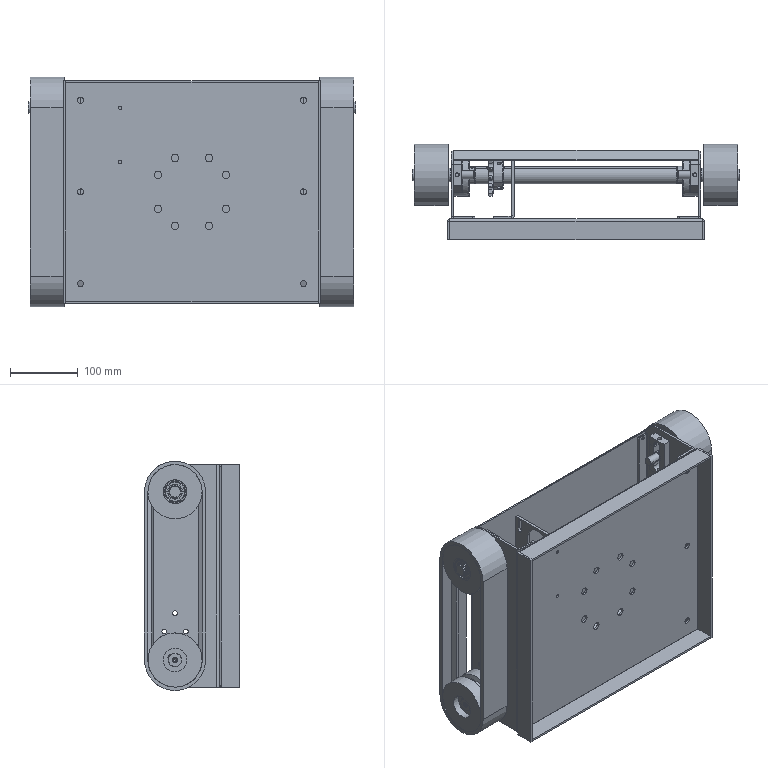Assembly | SolidWorks | mm | 25 component files | 27 solids | 1237 faces | box 483 x 140 x 338 mm | volume 2614208 mm3 | cylinder 515 | plane 353 | cone 163 | torus 156 | spline 50 | commonest cylinder face diameters 5 x28 80 x28 7 x26 35 x24 9 x21 17 x20 1 x18 20 x18
Bill of materials:
CCD02LiftingBasePlate | 1 |  | Shallow rectangular tray-like plate: thin flat rectangular panel with a narrow flange turned up along the perimeter, pierced by a hole pattern.
CCD03BearingSupportPlate | 1 |  | Long bent sheet bracket with a flanged channel-type profile: a main web with rounded corners at one end, a side flange with slotted holes, and short return flanges.
CCD04BearingSupportPlateA | 1 |  | Long bent sheet bracket, roughly a mirror version of the previous bracket: a web with a long slot, a triangular small-hole group and a large hole, a slotted side flange, plus an extra narrow flange and a raised tab near the top.
CCD06DriveWheel | 2 |  | Cylindrical grooved wheel or pulley-like disc with one central circumferential V-shaped groove and a central bore with a keyway.
CCD07DriveAxis | 1 |  | Long slender stepped round shaft: a larger central section with smaller stepped diameters toward both ends.
CCD08Anti-slipBelt | 2 |  | Thin-walled closed obround (stadium-shaped) band or sleeve with straight sides and semicircular ends, open on both faces.
CCD09DriveSprocket | 1 |  | Toothed sprocket-like wheel with a single row of teeth and an integral cylindrical hub on one side, a keyed central bore, and radial holes in the hub.
CCD05DrivenWheel | 2 |  | Cylindrical grooved wheel similar to unnamed part: one central circumferential groove with angled sidewalls and a plain round central bore with no keyway.
CCD11TensioningAxis | 2 |  | Stepped cylindrical pin or short shaft: a long main body with a narrow circumferential groove near one end, a raised collar, and a reduced-diameter section with flats and a cross hole, ending in a smaller-diameter plain end.
CCD6003ZZ | 4 |  | Annular ring assembly-like body: an outer cylindrical ring and an inner ring of equal width, with a recessed annular face between them. It resembles a sealed or shielded rolling bearing envelope.
CCDAxisCard15 | 2 |  | Thin flat open ring with a split gap and two lugs, each with a round hole, at the open ends. Its shape resembles an external retaining ring.
CCD12DriveWheelRetainingRing | 2 |  | Flat circular washer-like disc with a central round hole and small chamfers on its outer and inner edges.
CCD13MotorPlate | 1 |  | L-shaped bent sheet/plate bracket with an inside corner radius. The larger leg has a large central obround (oval) cutout and four straight slots, two near each side edge, running along the leg's height. The shorter leg has two slots running across it, one near each end.
CCD15ChainCover | 1 |  | Thin rectangular flat panel with four small round holes, one near each corner. Two opposite edges are bent into short, shallow angled flanges that turn the same way, giving a shallow tray-like edge profile.
CCDUCFB204 | 2 | AISI 1045 Steel, Cold Drawn | Compact housing with a flat mounting plate shaped like a pointed or triangular tab, carrying three round through-holes. A short web or rib joins the plate to an offset cylindrical boss. The boss holds a concentric ring insert with a central bore and an extended collar that sticks out on one side. A small nipple-like protrusion is on the outer rim of the boss, and a small round feature is on the collar.
Mates:
1. coincident | CCD02LiftingBasePlate-1 edge at (46.879, 42.251, -110) dir (0, 1, 0) r 4.5 | CCD03BearingSupportPlate-1 sketch segment at (46.879, 42.251, -110) dir (0, -1, 0) r 4.5
2. concentric | CCD02LiftingBasePlate-1 face at (46.879, 32.251, -110) dir (0, 1, 0) r 4.5 | CCD03BearingSupportPlate-1 sketch segment at (46.879, 42.251, -110) dir (0, -1, 0) r 4.5
3. concentric | CCD02LiftingBasePlate-1 face at (46.879, 32.251, 160) dir (0, 1, 0) r 4.5 | CCD03BearingSupportPlate-1 sketch segment at (46.879, 42.251, 160) dir (0, -1, 0) r 4.5
4. concentric | CCD02LiftingBasePlate-1 face at (-281.121, 32.251, -110) dir (0, 1, 0) r 4.5 | CCD04BearingSupportPlateA-1 sketch segment at (-281.121, 42.251, -110) dir (0, -1, 0) r 4.25
5. concentric | CCD02LiftingBasePlate-1 face at (-281.121, 32.251, 160) dir (0, 1, 0) r 4.5 | CCD04BearingSupportPlateA-1 sketch segment at (-281.121, 42.251, 160) dir (0, -1, 0) r 4.25
6. coincident | CCD02LiftingBasePlate-1 face at (-306.121, 42.251, -139) dir (0, 1, 0) | CCD04BearingSupportPlateA-1 face at (-301.121, 42.251, -139) dir (0, -1, 0)
7. coincident | CCD04BearingSupportPlateA-1 face at (-298.121, 42.251, -139) dir (1, 0, 0) | CCDUCFB204-1 face at (-298.121, 107.251, -99) dir (-1, 0, 0)
8. concentric | CCD04BearingSupportPlateA-1 face at (-291.121, 107.251, -99) dir (-1, 0, 0) r 15 | CCDUCFB204-1 face at (-266.321, 107.251, -99) dir (-1, 0, 0) r 10
9. concentric | CCD04BearingSupportPlateA-1 face at (-301.121, 123.251, -57) dir (-1, 0, 0) r 3.4 | CCDUCFB204-1 face at (-285.121, 123.251, -57) dir (-1, 0, 0) r 4.75
10. coincident | CCD03BearingSupportPlate-1 face at (63.879, 42.251, -139) dir (-1, 0, 0) | CCDUCFB204-2 face at (63.879, 107.251, -99) dir (1, 0, 0)
11. concentric | CCD03BearingSupportPlate-1 face at (73.879, 107.251, -99) dir (-1, 0, 0) r 15 | CCDUCFB204-2 face at (32.079, 107.251, -99) dir (1, 0, 0) r 10
12. concentric | CCD03BearingSupportPlate-1 face at (63.879, 123.251, -57) dir (-1, 0, 0) r 3.4 | CCDUCFB204-2 face at (50.879, 123.251, -57) dir (1, 0, 0) r 4.75
13. distance | CCD06DriveWheel-1 face at (-306.121, 107.251, -99) dir (1, 0, 0) | CCD04BearingSupportPlateA-1 face at (-301.121, 42.251, -139) dir (-1, 0, 0)
14. distance | CCD06DriveWheel-11 face at (71.879, 107.251, -99) dir (-1, 0, 0) | CCD03BearingSupportPlate-1 face at (66.879, 42.251, -139) dir (1, 0, 0)
15. concentric | CCDUCFB204-2 face at (32.079, 107.251, -99) dir (1, 0, 0) r 10 | CCD06DriveWheel-11 face at (119.879, 107.251, -99) dir (1, 0, 0) r 8.5
16. concentric | CCDUCFB204-1 face at (-266.321, 107.251, -99) dir (-1, 0, 0) r 10 | CCD06DriveWheel-1 face at (-356.521, 107.251, -99) dir (1, 0, 0) r 40
17. concentric | CCDUCFB204-1 face at (-266.321, 107.251, -99) dir (-1, 0, 0) r 10 | CCD07DriveAxis-1 face at (-453.536, 107.251, -99) dir (-1, 0, 0) r 10
18. coincident | CCD06DriveWheel-1 face at (-344.121, 107.251, -99) dir (-1, 0, 0) | CCD07DriveAxis-1 face at (-344.121, 107.251, -99) dir (-1, 0, 0)
19. coincident | CCD06DriveWheel-1 face at (-354.121, 112.278, -92.145) dir (0, 0.5458, -0.8379) | CCD07DriveAxis-1 face at (-344.121, 110.055, -93.593) dir (0, 0.5458, -0.8379)
20. coincident | CCD06DriveWheel-11 face at (119.879, 115.553, -97.173) dir (0, -0.5458, 0.8379) | CCD07DriveAxis-1 face at (109.879, 113.33, -98.621) dir (0, -0.5458, 0.8379)
21. concentric | CCD06DriveWheel-1 face at (-356.521, 107.251, -99) dir (1, 0, 0) r 40 | CCD08Anti-slipBelt-1 face at (-305.121, 107.251, -99) dir (-1, 0, 0) r 40
22. distance | CCD08Anti-slipBelt-1 face at (-355.121, 107.251, -99) dir (-1, 0, 0) | CCD06DriveWheel-1 face at (-354.121, 107.251, -99) dir (-1, 0, 0)
23. concentric | CCD06DriveWheel-11 face at (122.279, 107.251, -99) dir (-1, 0, 0) r 40 | CCD08Anti-slipBelt-2 face at (120.879, 107.251, -99) dir (-1, 0, 0) r 40
24. concentric | CCD07DriveAxis-1 face at (-453.536, 107.251, -99) dir (-1, 0, 0) r 12.5 | CCD09DriveSprocket-1 face at (-224.321, 107.251, -99) dir (-1, 0, 0) r 12.5
25. distance | CCD09DriveSprocket-1 face at (-246.321, 127.838, -85.589) dir (-1, 0, 0) | CCDUCFB204-1 face at (-266.321, 107.251, -99) dir (1, 0, 0)
26. coincident | CCD07DriveAxis-1 face at (-246.121, 113.406, -91.41) dir (0, 0.5458, -0.8379) | CCD09DriveSprocket-1 face at (-247.267, 118.434, -88.135) dir (0, 0.5458, -0.8379)
27. concentric | CCD04BearingSupportPlateA-1 sketch segment at (-301.121, 107.251, 149) dir (-1, 0, 0) r 6.25 | CCD11-00TensioningAssembly-1/CCD11TensioningAxis-1 face at (-440.877, 107.251, 149) dir (-1, 0, 0) r 10
28. coincident | CCD04BearingSupportPlateA-1 face at (-301.121, 42.251, -139) dir (-1, 0, 0) | CCD11-00TensioningAssembly-1/CCD11TensioningAxis-1 face at (-301.121, 107.251, 149) dir (1, 0, 0)
29. parallel | CCD04BearingSupportPlateA-1 face at (-301.121, 101.001, 169) dir (0, 1, 0) | CCD11-00TensioningAssembly-1/CCD11TensioningAxis-1 face at (-301.121, 101.251, 159.031) dir (0, -1, 0)
30. coincident | CCD03BearingSupportPlate-1 face at (66.879, 42.251, -139) dir (1, 0, 0) | CCD11-00TensioningAssembly-2/CCD11TensioningAxis-1 face at (66.879, 107.251, 149) dir (-1, 0, 0)
31. concentric | CCD11-00TensioningAssembly-1/CCD05DrivenWheel-1 face at (-483.663, 107.251, 149) dir (-1, 0, 0) r 40 | CCD11-00TensioningAssembly-2/CCD05DrivenWheel-1 face at (249.421, 107.251, 149) dir (1, 0, 0) r 40
32. concentric | CCD03BearingSupportPlate-1 face at (57.879, 107.251, 179) dir (0, 0, 1) r 3.1 | CCD11-00TensioningAssembly-2/CCD11TensioningAxis-1 face at (57.879, 107.251, 141.5) dir (0, 0, -1) r 2.5
33. concentric | CCD06DriveWheel-1 face at (-356.521, 107.251, -99) dir (1, 0, 0) r 40 | CCD12DriveWheelRetainingRing-1 face at (-344.121, 107.251, -99) dir (-1, 0, 0) r 10
34. coincident | CCD07DriveAxis-1 face at (-344.121, 107.251, -99) dir (-1, 0, 0) | CCD12DriveWheelRetainingRing-1 face at (-344.121, 107.251, -99) dir (1, 0, 0)
35. concentric | CCD06DriveWheel-11 face at (122.279, 107.251, -99) dir (-1, 0, 0) r 40 | CCD12DriveWheelRetainingRing-2 face at (109.879, 107.251, -99) dir (1, 0, 0) r 10
36. coincident | CCD07DriveAxis-1 face at (109.879, 111.891, -106.122) dir (1, 0, 0) | CCD12DriveWheelRetainingRing-2 face at (109.879, 107.251, -99) dir (-1, 0, 0)
37. coincident | CCD02LiftingBasePlate-1 face at (-306.121, 42.251, -139) dir (0, 1, 0) | CCD13MotorPlate-1 face at (-212.121, 42.251, 59) dir (0, -1, 0)
38. concentric | CCD02LiftingBasePlate-1 face at (-223.121, 42.251, 149) dir (0, 1, 0) r 2.5 | CCD13MotorPlate-1 sketch segment at (-223.121, 46.251, 149) dir (0, 1, 0) r 3.5
39. coincident | CCD04BearingSupportPlateA-1 face at (-301.121, 142.251, -139) dir (0, 1, 0) | CCD15ChainCover-1 face at (-297.121, 142.251, 175) dir (0, -1, 0)
40. concentric | CCD03BearingSupportPlate-1 face at (54.879, 142.251, -115) dir (0, 1, 0) r 2.5 | CCD15ChainCover-1 face at (54.879, 133.451, -115) dir (0, 1, 0) r 3.5
41. concentric | CCD04BearingSupportPlateA-1 face at (-289.121, 142.251, 165) dir (0, 1, 0) r 2.5 | CCD15ChainCover-1 face at (-289.121, 133.451, 165) dir (0, 1, 0) r 3.5
42. concentric | CCD11TensioningAxis-1 face at (-216.169, -13.326, 0) dir (-1, 0, 0) r 8.5 | CCD05DrivenWheel-1 face at (-258.955, -13.326, 0) dir (-1, 0, 0) r 17.5
43. coincident | CCD11TensioningAxis-1 face at (-81.413, -4.826, 0) dir (-1, 0, 0) | CCD05DrivenWheel-1 face at (-81.413, 26.644, -1.568) dir (1, 0, 0)
44. coincident | CCD05DrivenWheel-1 face at (-129.413, 4.161, -0.6862) dir (-1, 0, 0) | CCD6003ZZ-1 face at (-129.413, 3.874, 0) dir (-1, 0, 0)
45. concentric | CCD05DrivenWheel-1 face at (-258.955, -13.326, 0) dir (-1, 0, 0) r 17.5 | CCD6003ZZ-1 face at (-129.414, -13.326, 0) dir (1, 0, 0) r 8.5
46. coincident | CCD05DrivenWheel-1 face at (-81.413, 26.644, -1.568) dir (1, 0, 0) | CCD6003ZZ-2 face at (-81.413, -6.758, -15.897) dir (1, 0, 0)
47. concentric | CCD11TensioningAxis-1 face at (-216.169, -13.326, 0) dir (-1, 0, 0) r 8.5 | CCD6003ZZ-2 face at (-81.412, -13.326, 0) dir (-1, 0, 0) r 17.5
48. coincident | CCD11TensioningAxis-1 face at (-129.413, -6.426, 0) dir (-1, 0, 0) | CCDAxisCard15-1 face at (-129.413, -23.226, -2.25) dir (1, 0, 0)
49. concentric | CCD11TensioningAxis-1 face at (-216.169, -13.326, 0) dir (-1, 0, 0) r 8.5 | CCDAxisCard15-1 face at (-130.413, -13.326, 0) dir (1, 0, 0) r 6.9